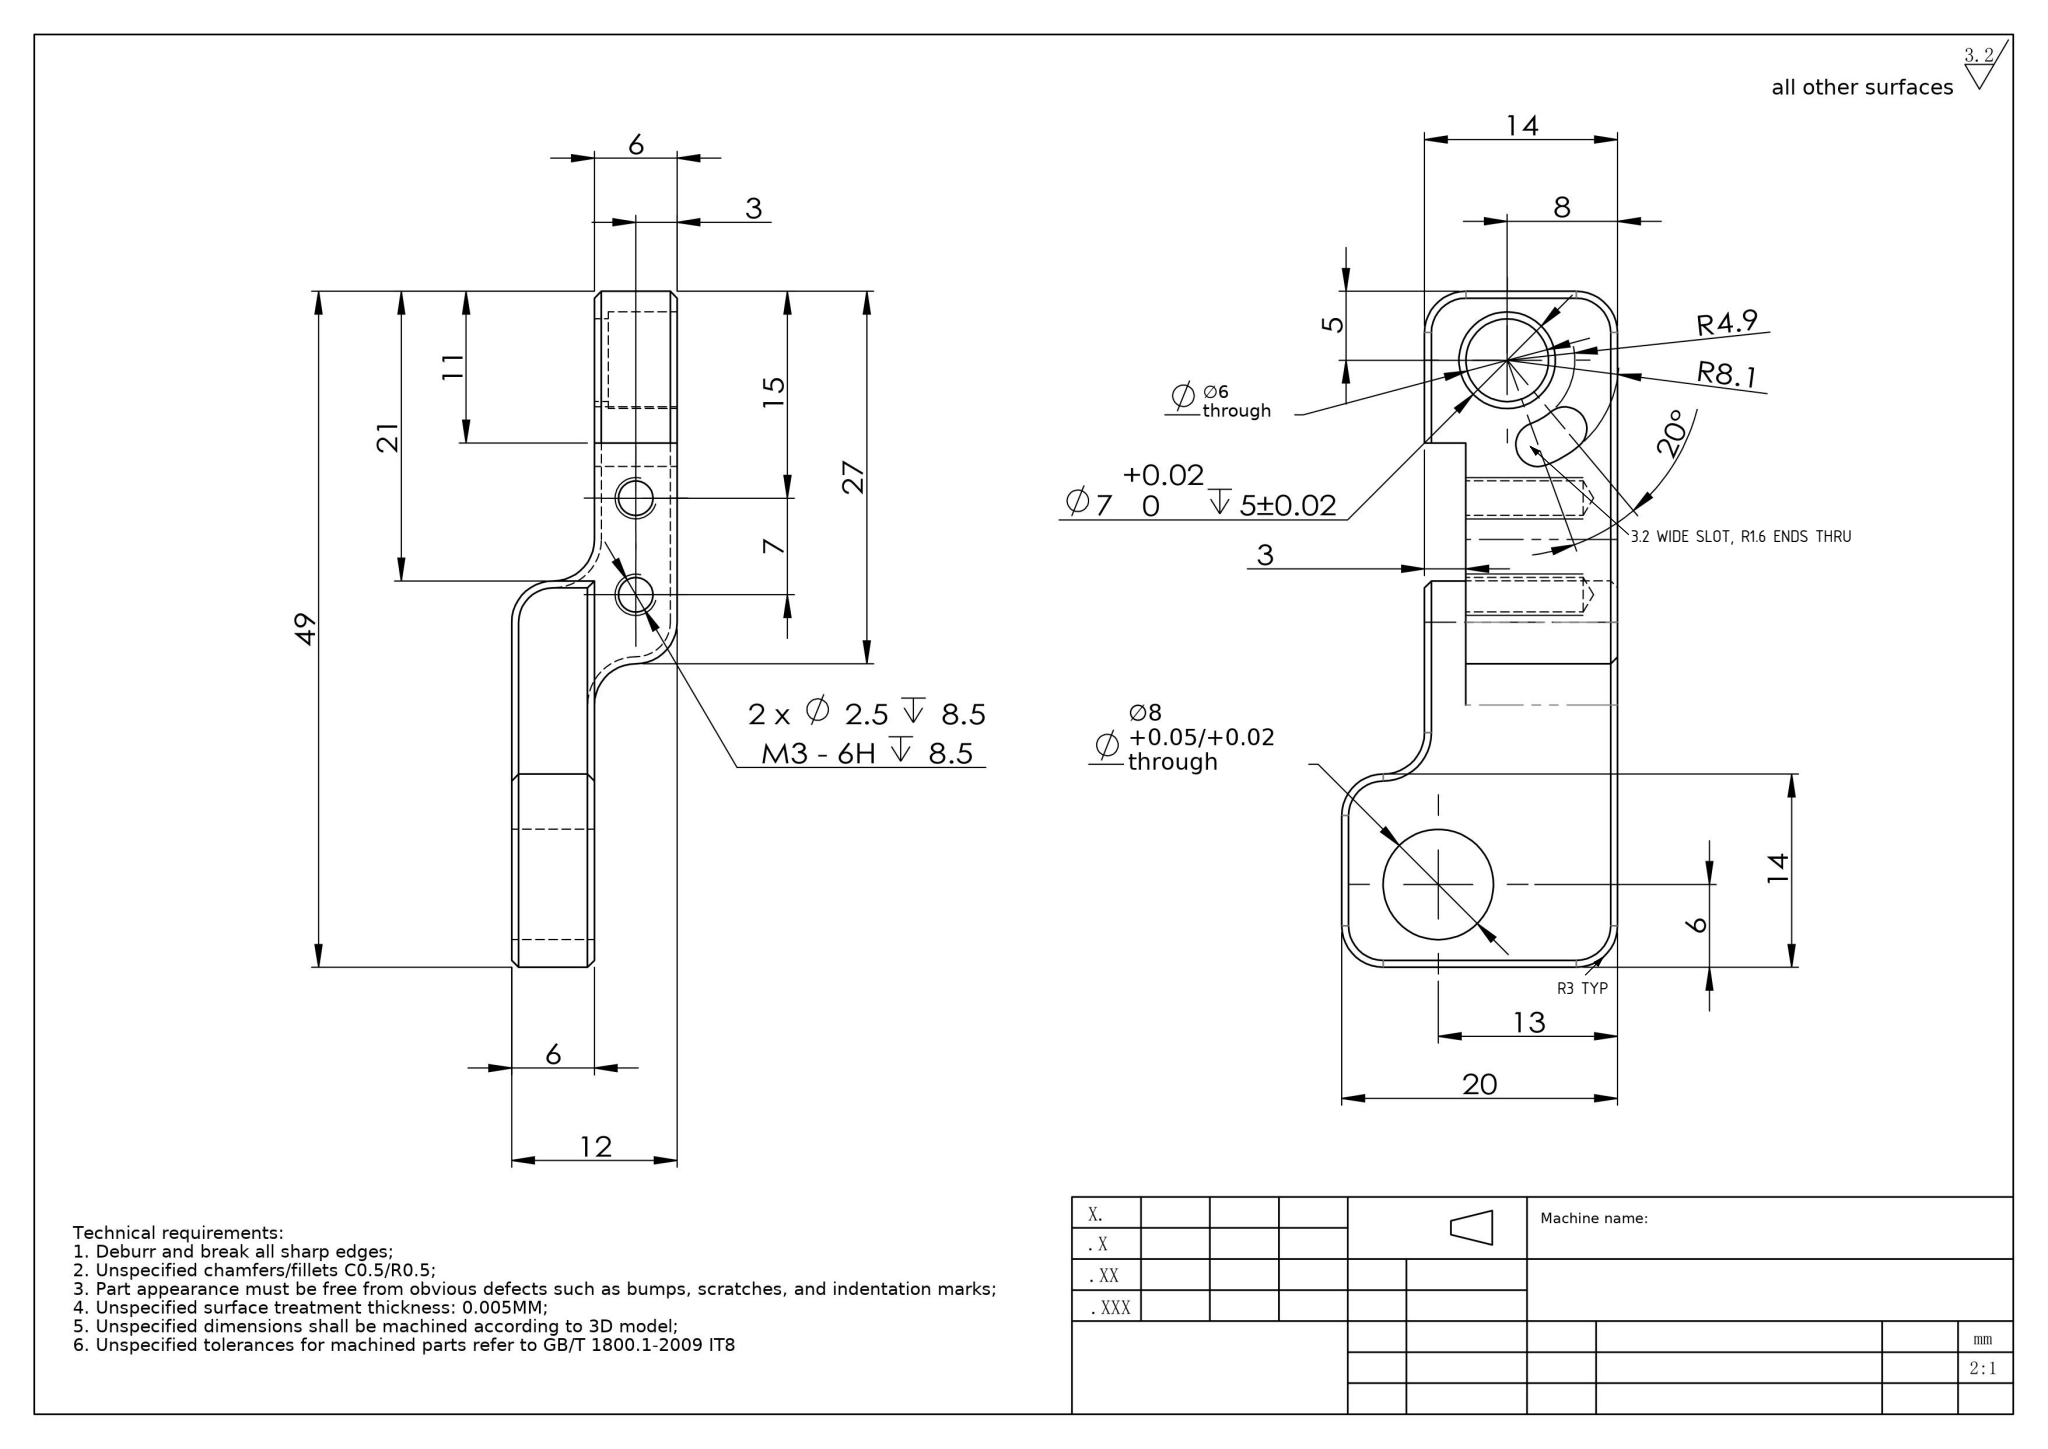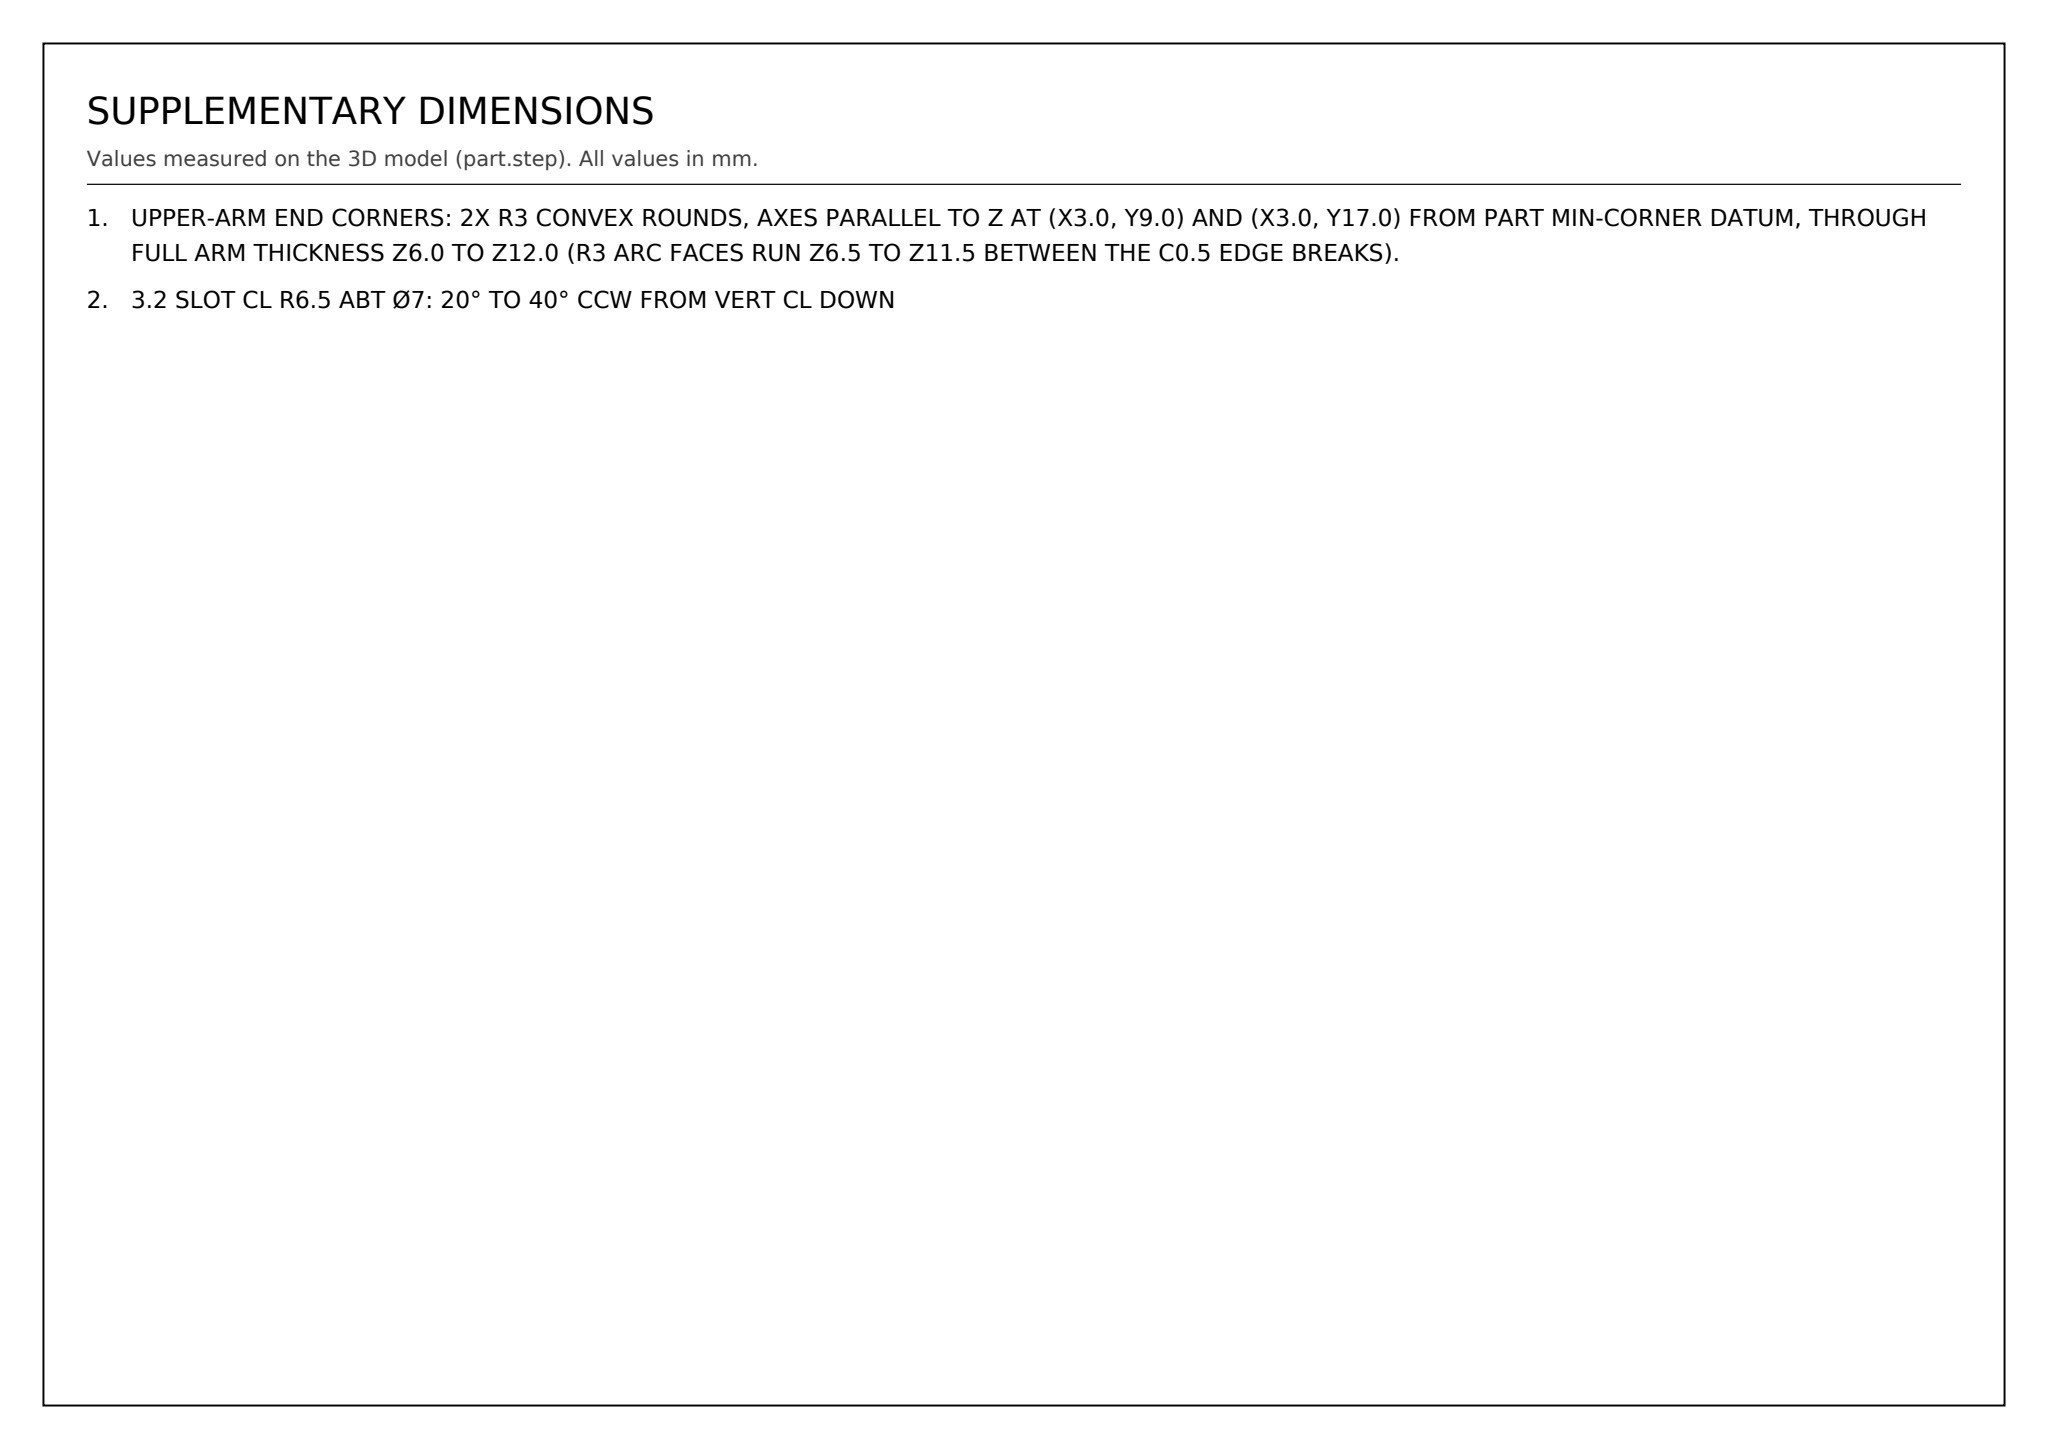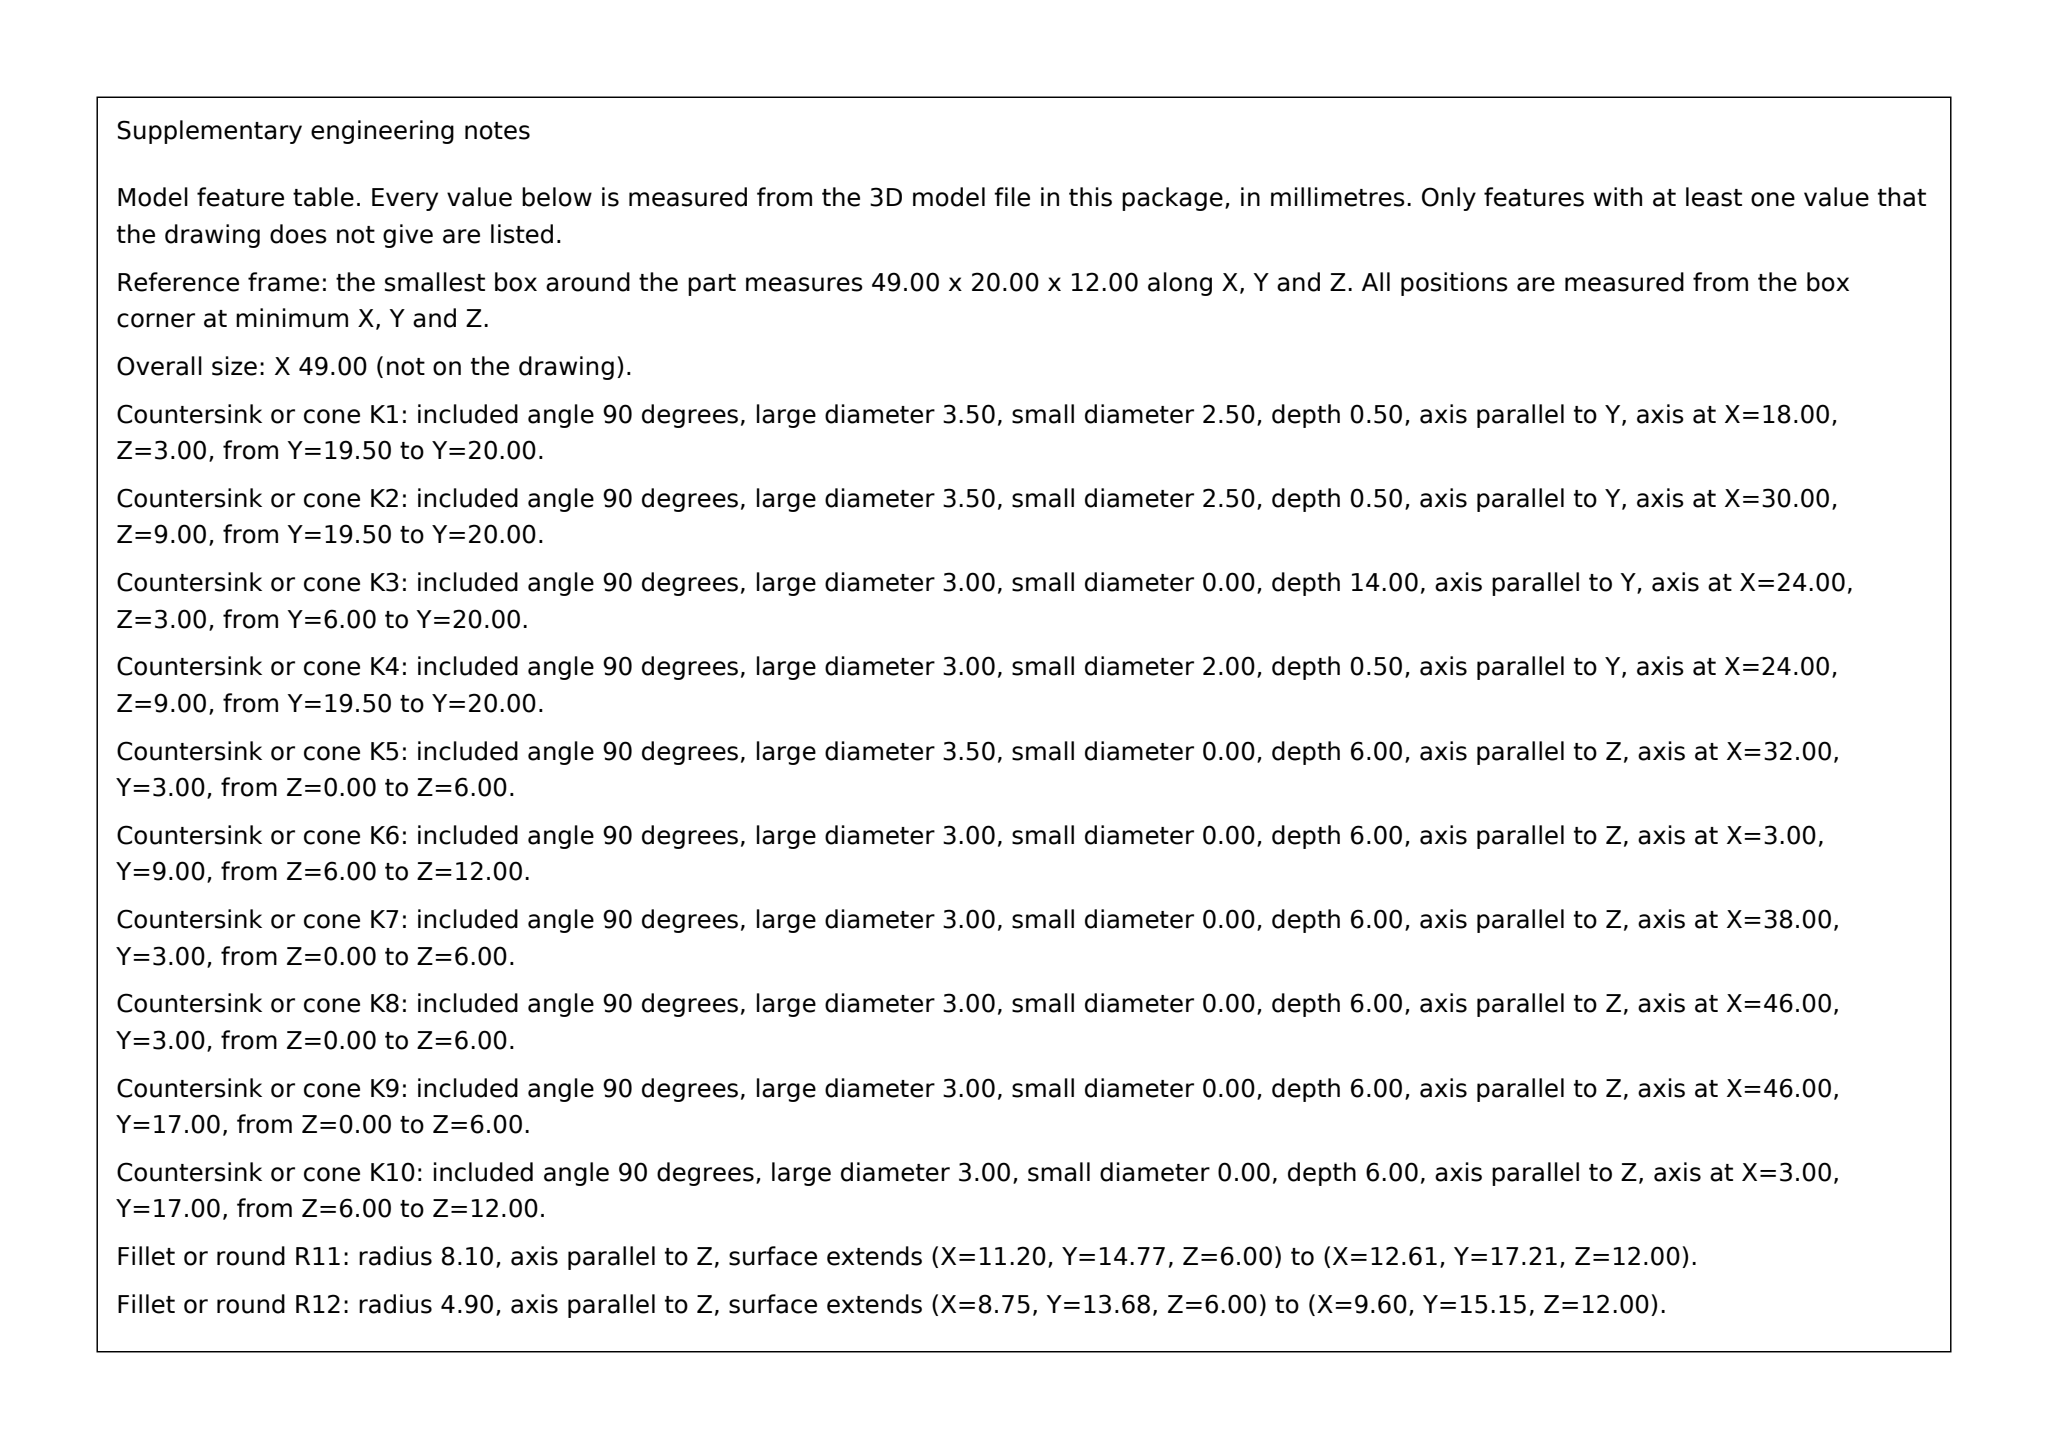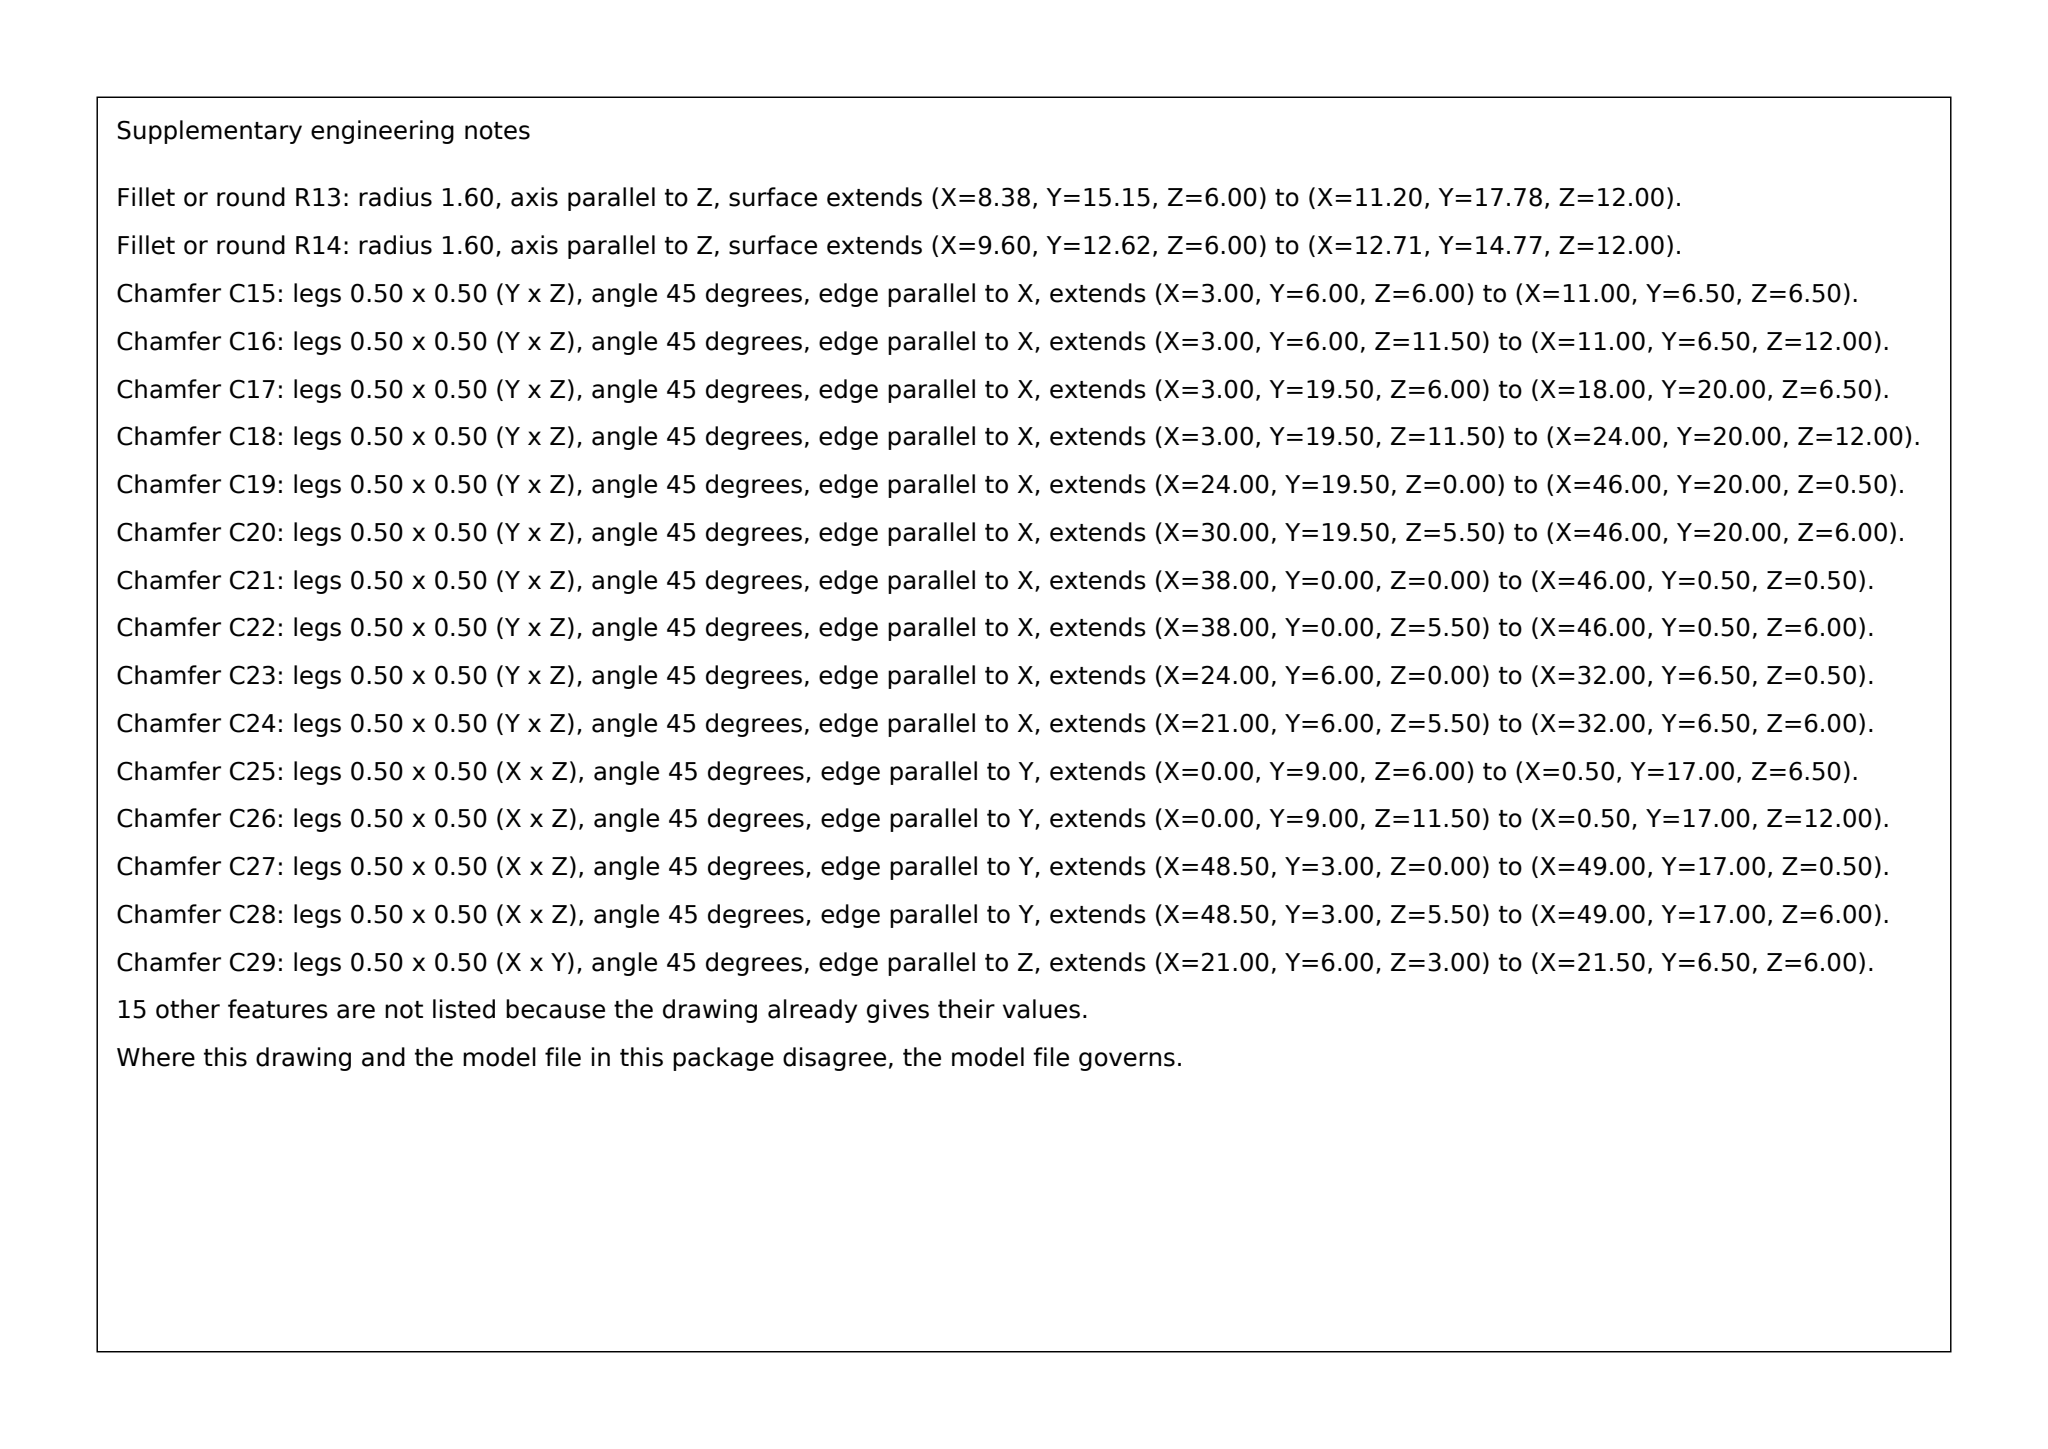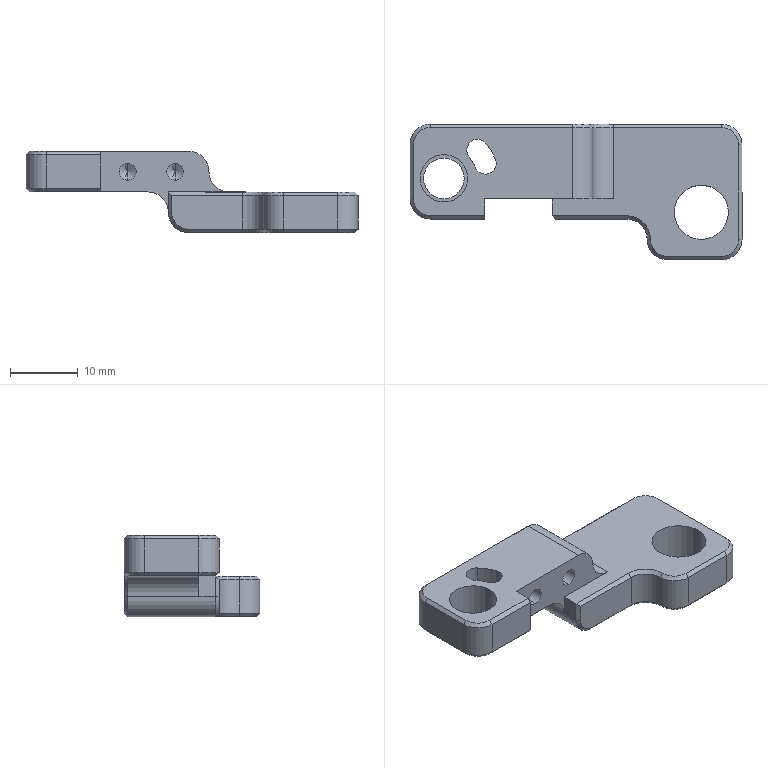Part | SolidWorks | mm | 1 solid | 75 faces | box 49 x 20 x 12 mm | volume 4053 mm3 | plane 29 | cylinder 25 | cone 21 | commonest cylinder face diameters 6 x12 2.5 x4 3.2 x3 8 x2 7 x2 16.2 x1 9.8 x1
Drawing notes:
RELIEF SLOT: 3.2 WIDE x R1.6 FULL-RADIUS ENDS, END CENTRES AT (X10.0, Y16.2) AND (X11.1, Y14.2) FROM PART MIN-CORNER DATUM (X0 = LEFT END FACE, Y0 = BACK FACE); THRU THE 6 THK ARM (Z6.0 TO Z12.0). | from the solid: cylinders: two 'concave arc' Ø3.2, axis z at [10.0,16.2] and [11.1,14.2], from 6.0 to 12.0, arc_deg 180
LOWER LOBE OUTER CORNERS: R3 TYP, ARC AXES (Z-DIR) AT X38.0/Y3.0, X46.0/Y3.0, X46.0/Y17.0; INNER RE-ENTRANT CORNER R3 AT X32.0/Y3.0; ALL THROUGH LOBE THICKNESS Z0.5 TO Z5.5. | from the solid: cylinders: convex arc Ø6.0 axis z at [38.0,3.0], [46.0,17.0], [46.0,3.0] and concave arc Ø6.0 axis z at [32.0,3.0], from 0.5 to 5.5, arc_deg 90
UPPER-ARM END CORNERS: 2X R3 CONVEX ROUNDS, AXES PARALLEL TO Z AT (X3.0, Y9.0) AND (X3.0, Y17.0) FROM PART MIN-CORNER DATUM, THROUGH FULL ARM THICKNESS Z6.0 TO Z12.0 (R3 ARC FACES RUN Z6.5 TO Z11.5 BETWEEN THE C0.5 EDGE BREAKS). | from the solid: cylinders: convex arc (round/outer radius) dia 6.0, axis z at [3.0, 9.0] and [3.0, 17.0], from 6.5 to 11.5, 90 deg each
3.2 SLOT CL R6.5 ABT Ø7: 20° TO 40° CCW FROM VERT CL DOWN | from the solid: Slot end arcs Ø3.2 at (10.0,16.2) and (11.1,14.2) vs Ø7 axis (5.0,12.0): radius 6.5, angles 40.0° and 19.8° from +x (downward vert in RH view); R4.9/R8.1 arcs 20° sweep about same axis